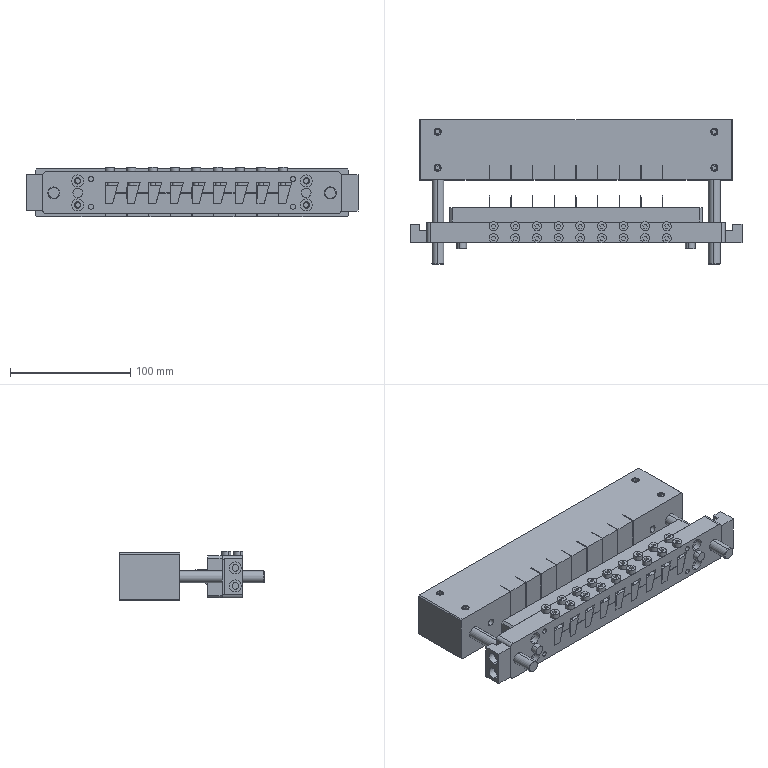Assembly | SolidWorks | mm | 49 component files | 49 solids | 1077 faces | box 276 x 120 x 41.5 mm | volume 758945 mm3 | plane 699 | cylinder 314 | cone 64 | commonest cylinder face diameters 4 x72 4.2 x52 6 x36 10 x36 7.5 x36 3.3 x18 2.5 x18 2 x18
Bill of materials:
20#EngravingKnifeBlade | 9 |  | Thin flat plate with an angled pointed end. It looks like a utility/craft knife blade.
6x30TPunch | 2 | Cr12 | Stepped cylindrical pin: a short larger-diameter collar/head and a longer smaller-diameter shaft.
8TC-A15004-60-26A | 1 | Cr12 | Long rectangular bar with holes near each end and a row of thin evenly spaced slits/lines across the middle section.
8TC-A15004-60-27A | 1 | Cr12 | Elongated rectangular bar with rounded edges, a row of tapered (trapezoidal) through-openings, and multiple hole patterns.
8TC-A15004-60-28A | 1 | Cr12 | Long flat rectangular bar with chamfered corners and three holes at each end.
8TC-A15004-60-30A | 2 | Chrome Plated Hard Rod | Slender cylindrical pin/shaft with two circumferential grooves near one end.
8TC-A15004-60-31A | 9 | #45 | Block with one inclined side face (trapezoidal side profile) and two round holes in the top face.
8TC-A15004-60-34B | 2 | #45 | Rectangular block with a rectangular step/notch cut from one top corner, giving an L-shaped profile, and two holes through one face.
M4x20HexSocketCapScrew | 18 | #45 | Shape like a socket head cap screw: cylindrical head with a hexagonal socket recess and a plain cylindrical shank.
M6x8GrubScrew | 4 | #45 | Short cylinder with a hexagonal socket in one end and a conical/chamfered point at the other. It looks like a cone-point set screw.
Mates:
1. concentric | 8TC-A15004-60-30A-2 face at (-88.286, 25, 0) dir (0, -1, 0) r 5 | 8TC-A15004-60-26A-1 face at (-88.286, 25, 0) dir (0, -1, 0) r 5
2. coincident | 8TC-A15004-60-30A-2 face at (-88.286, 25, 0) dir (0, 1, 0) | 8TC-A15004-60-26A-1 face at (26.714, 25, 0) dir (0, 1, 0)
3. concentric | 8TC-A15004-60-26A-1 face at (141.714, 25, 0) dir (0, -1, 0) r 5 | 8TC-A15004-60-30A-1 face at (141.714, 25, 0) dir (0, -1, 0) r 5
4. coincident | 8TC-A15004-60-26A-1 face at (26.714, 25, 0) dir (0, 1, 0) | 8TC-A15004-60-30A-1 face at (141.714, 25, 0) dir (0, 1, 0)
5. distance | 8TC-A15004-60-27A-1 face at (26.714, -60, 0) dir (0, 1, 0) | 8TC-A15004-60-26A-1 face at (26.714, -25, 0) dir (0, -1, 0)
6. coincident | 8TC-A15004-60-26A-1 plane at (26.714, 0, 0) dir (0, 1, 0) | assembly plane at (0, 0, 0) dir (0, 1, 0)
7. coincident | 8TC-A15004-60-26A-1 plane at (26.714, 0, 0) dir (0, 0, -1) | assembly plane at (0, 0, 0) dir (0, 0, 1)
8. coincident | 8TC-A15004-60-26A-1 face at (156.714, 25, 20) dir (0, 0, 1) | M6x8GrubScrew-1 face at (141.714, -15, 20) dir (0, 0, 1)
9. concentric | 8TC-A15004-60-26A-1 face at (141.714, -15, 20) dir (0, 0, 1) r 3 | M6x8GrubScrew-1 face at (141.714, -15, 12) dir (0, 0, -1) r 3
10. concentric | 8TC-A15004-60-26A-1 face at (141.714, 15, 20) dir (0, 0, 1) r 3 | M6x8GrubScrew-2 face at (141.714, 15, 12) dir (0, 0, -1) r 3
11. coincident | M6x8GrubScrew-1 face at (141.714, -15, 20) dir (0, 0, 1) | M6x8GrubScrew-2 face at (141.714, 15, 20) dir (0, 0, 1)
12. concentric | 8TC-A15004-60-26A-1 face at (-88.286, 15, 20) dir (0, 0, 1) r 3 | M6x8GrubScrew-3 face at (-88.286, 15, 12) dir (0, 0, -1) r 3
13. coincident | 8TC-A15004-60-26A-1 face at (156.714, 25, 20) dir (0, 0, 1) | M6x8GrubScrew-3 face at (-88.286, 15, 20) dir (0, 0, 1)
14. concentric | 8TC-A15004-60-26A-1 face at (-88.286, -15, 20) dir (0, 0, 1) r 3 | M6x8GrubScrew-4 face at (-88.286, -15, 12) dir (0, 0, -1) r 3
15. coincident | M6x8GrubScrew-3 face at (-88.286, 15, 20) dir (0, 0, 1) | M6x8GrubScrew-4 face at (-88.286, -15, 20) dir (0, 0, 1)
16. concentric | 8TC-A15004-60-27A-1 face at (102.214, -73.5, 17.5) dir (0, 0, 1) r 2 | M4x20HexSocketCapScrew-18 face at (102.214, -73.5, -2.5) dir (0, 0, -1) r 2
17. concentric | 8TC-A15004-60-27A-1 face at (102.214, -63.5, 17.5) dir (0, 0, 1) r 2 | M4x20HexSocketCapScrew-1 face at (102.214, -63.5, -2.5) dir (0, 0, -1) r 2
18. coincident | 8TC-A15004-60-27A-1 face at (150.714, -60, 17.5) dir (0, 0, 1) | M4x20HexSocketCapScrew-18 face at (105.678, -72.064, 17.5) dir (0, 0, -1)
19. coincident | 8TC-A15004-60-27A-1 face at (150.714, -60, 17.5) dir (0, 0, 1) | M4x20HexSocketCapScrew-1 face at (105.678, -62.064, 17.5) dir (0, 0, -1)
20. coincident | 8TC-A15004-60-27A-1 face at (98.514, -60, 4.75) dir (1, 0, 0) | 20#EngravingKnifeBlade-1 face at (98.514, -4652.617, 846.55) dir (-1, 0, 0)
21. coincident | 8TC-A15004-60-27A-1 face at (26.714, -60, 0) dir (0, 1, 0) | 20#EngravingKnifeBlade-1 edge at (98.914, -60, 4.5) dir (-1, 0, 0)
22. width | 8TC-A15004-60-31A-1 face at (101.714, -60, 6) dir (0, 1, 0) | 8TC-A15004-60-31A-1 face at (101.714, -77, 6) dir (0, -1, 0) | 8TC-A15004-60-27A-1 face at (26.714, -60, 0) dir (0, 1, 0) | 8TC-A15004-60-27A-1 face at (26.714, -77, 0) dir (0, -1, 0)
23. coincident | 8TC-A15004-60-27A-1 face at (98.714, -60, -9) dir (1, 0, 0) | 8TC-A15004-60-31A-1 face at (98.714, -77, 6) dir (-1, 0, 0)
24. coincident | 8TC-A15004-60-27A-1 face at (104.714, -60, -9) dir (0, 0, 1) | 8TC-A15004-60-31A-1 face at (98.714, -77, -9) dir (0, 0, -1)
25. width | 20#EngravingKnifeBlade-1 face at (98.914, -59, 4.5) dir (0, 0, 1) | 20#EngravingKnifeBlade-1 face at (98.914, -77, -4.5) dir (0, 0, -1) | 8TC-A15004-60-27A-1 face at (98.914, -60, -4.75) dir (0, 0, 1) | 8TC-A15004-60-27A-1 face at (98.914, -60, 4.75) dir (0, 0, -1)
26. concentric | 8TC-A15004-60-27A-1 face at (-88.286, -60, 0) dir (0, -1, 0) r 5 | 8TC-A15004-60-30A-2 face at (-88.286, 25, 0) dir (0, -1, 0) r 5
27. parallel | 8TC-A15004-60-27A-1 face at (150.714, -60, 17.5) dir (0, 0, 1) | 20#EngravingKnifeBlade-1 face at (98.914, -77, -4.5) dir (0, 0, -1)
28. coincident | 8TC-A15004-60-27A-1 face at (26.714, -60, 0) dir (0, 1, 0) | 8TC-A15004-60-28A-2 face at (26.714, -60, 0) dir (0, -1, 0)
29. concentric | 8TC-A15004-60-27A-1 face at (121.714, -60, 0) dir (0, -1, 0) r 3 | 8TC-A15004-60-28A-2 face at (121.714, -68, 0) dir (0, 1, 0) r 3
30. concentric | 8TC-A15004-60-27A-1 face at (-68.286, -60, 0) dir (0, -1, 0) r 3 | 8TC-A15004-60-28A-2 face at (-68.286, -68, 0) dir (0, 1, 0) r 3
31. concentric | 8TC-A15004-60-27A-1 face at (-68.286, -60, 0) dir (0, -1, 0) r 3 | 6x30TPunch-1 face at (-68.286, -77, 0) dir (0, 1, 0) r 3
32. coincident | 8TC-A15004-60-27A-1 face at (26.714, -77, 0) dir (0, -1, 0) | 6x30TPunch-1 face at (-68.286, -77, 0) dir (0, 1, 0)
33. coincident | 8TC-A15004-60-27A-1 face at (26.714, -77, 0) dir (0, -1, 0) | 6x30TPunch-2 face at (121.714, -77, 0) dir (0, 1, 0)
34. concentric | 8TC-A15004-60-27A-1 face at (121.714, -60, 0) dir (0, -1, 0) r 3 | 6x30TPunch-2 face at (121.714, -77, 0) dir (0, 1, 0) r 3
35. coincident | 8TC-A15004-60-27A-1 face at (-97.286, -60, -17.5) dir (-1, 0, 0) | 8TC-A15004-60-34B-1 face at (-97.286, -69.5, 0) dir (1, 0, 0)
36. coincident | 8TC-A15004-60-27A-1 face at (26.714, -77, 0) dir (0, -1, 0) | 8TC-A15004-60-34B-1 face at (-111.286, -77, -15) dir (0, -1, 0)
37. coincident | 8TC-A15004-60-27A-1 face at (150.714, -60, -17.5) dir (1, 0, 0) | 8TC-A15004-60-34B-3 face at (150.714, -69.5, -0.04597) dir (-1, 0, 0)
38. coincident | 8TC-A15004-60-27A-1 face at (26.714, -77, 0) dir (0, -1, 0) | 8TC-A15004-60-34B-3 face at (164.714, -77, 14.954) dir (0, -1, 0)
39. width | 8TC-A15004-60-34B-1 face at (-111.286, -62, -15) dir (0, 0, -1) | 8TC-A15004-60-34B-1 face at (-111.286, -62, 15) dir (0, 0, 1) | 8TC-A15004-60-27A-1 face at (150.714, -60, 17.5) dir (0, 0, 1) | 8TC-A15004-60-27A-1 face at (150.714, -60, -17.5) dir (0, 0, -1)